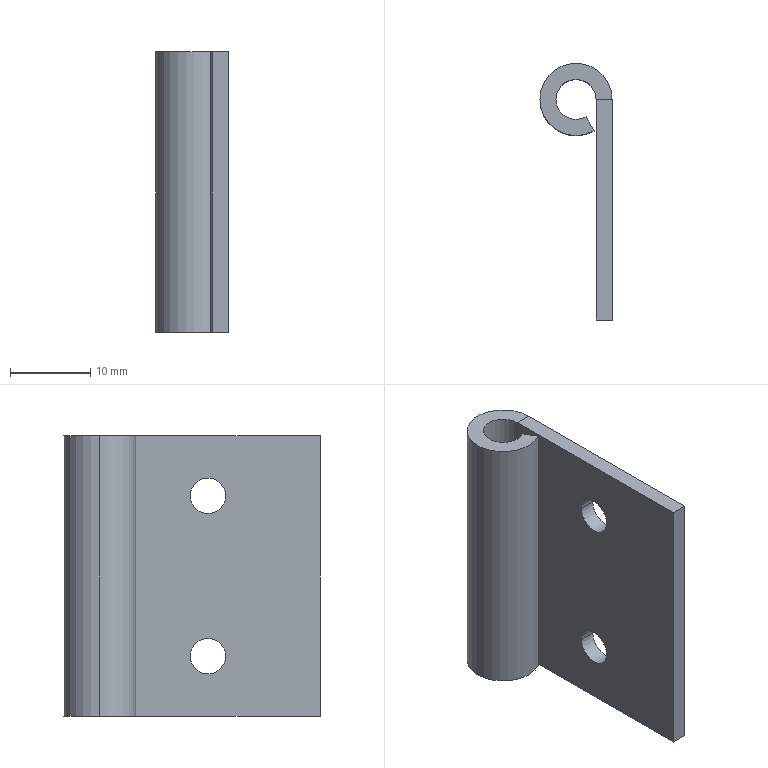Component | SolidWorks | FrontMiddleLowerDoor-1_Hinge(WeldedDoor)-1 | 1 solid | 16 faces | box 9 x 32 x 35 mm | volume 3146 mm3 | cylinder 8 | plane 8 | commonest cylinder face diameters 4.42 x4 9 x2 5 x2
STEP:
#1=CARTESIAN_POINT('',(16.299,14.851,-29.547));
#2=VERTEX_POINT('',#1);
#3=CARTESIAN_POINT('',(16.299,14.677,-29.547));
#4=VERTEX_POINT('',#3);
#5=CARTESIAN_POINT('',(16.299,14.764,-29.547));
#6=DIRECTION('',(1.,0.,-0.));
#7=DIRECTION('',(0.,1.,0.));
#8=AXIS2_PLACEMENT_3D('',#5,#6,#7);
#9=CIRCLE('',#8,0.087);
#10=EDGE_CURVE('',#2,#4,#9,.T.);
#11=ORIENTED_EDGE('',*,*,#10,.F.);
#12=CARTESIAN_POINT('',(16.378,14.851,-29.547));
#13=VERTEX_POINT('',#12);
#14=CARTESIAN_POINT('',(16.299,14.851,-29.547));
#15=DIRECTION('',(1.,0.,-0.));
#16=VECTOR('',#15,39.37);
#17=LINE('',#14,#16);
#18=EDGE_CURVE('',#2,#13,#17,.T.);
#19=ORIENTED_EDGE('',*,*,#18,.T.);
#20=CARTESIAN_POINT('',(16.378,14.677,-29.547));
#21=VERTEX_POINT('',#20);
#22=CARTESIAN_POINT('',(16.378,14.764,-29.547));
#23=DIRECTION('',(1.,0.,-0.));
#24=DIRECTION('',(0.,1.,0.));
#25=AXIS2_PLACEMENT_3D('',#22,#23,#24);
#26=CIRCLE('',#25,0.087);
#27=EDGE_CURVE('',#13,#21,#26,.T.);
#28=ORIENTED_EDGE('',*,*,#27,.T.);
#29=CARTESIAN_POINT('',(16.299,14.677,-29.547));
#30=DIRECTION('',(1.,0.,-0.));
#31=VECTOR('',#30,39.37);
#32=LINE('',#29,#31);
#33=EDGE_CURVE('',#4,#21,#32,.T.);
#34=ORIENTED_EDGE('',*,*,#33,.F.);
#35=EDGE_LOOP('',(#11,#19,#28,#34));
#36=FACE_OUTER_BOUND('',#35,.T.);
#37=CARTESIAN_POINT('',(16.299,14.764,-29.547));
#38=DIRECTION('',(1.,0.,-0.));
#39=DIRECTION('',(0.,-1.,0.));
#40=AXIS2_PLACEMENT_3D('',#37,#38,#39);
#41=CYLINDRICAL_SURFACE('',#40,0.087);
#42=ADVANCED_FACE('',(#36),#41,.F.);
#43=CARTESIAN_POINT('',(16.299,14.851,-30.335));
#44=VERTEX_POINT('',#43);
#45=CARTESIAN_POINT('',(16.299,14.677,-30.335));
#46=VERTEX_POINT('',#45);
#47=CARTESIAN_POINT('',(16.299,14.764,-30.335));
#48=DIRECTION('',(1.,0.,-0.));
#49=DIRECTION('',(0.,-1.,0.));
#50=AXIS2_PLACEMENT_3D('',#47,#48,#49);
#51=CIRCLE('',#50,0.087);
#52=EDGE_CURVE('',#44,#46,#51,.T.);
#53=ORIENTED_EDGE('',*,*,#52,.F.);
#54=CARTESIAN_POINT('',(16.378,14.851,-30.335));
#55=VERTEX_POINT('',#54);
#56=CARTESIAN_POINT('',(16.299,14.851,-30.335));
#57=DIRECTION('',(1.,0.,-0.));
#58=VECTOR('',#57,39.37);
#59=LINE('',#56,#58);
#60=EDGE_CURVE('',#44,#55,#59,.T.);
#61=ORIENTED_EDGE('',*,*,#60,.T.);
#62=CARTESIAN_POINT('',(16.378,14.677,-30.335));
#63=VERTEX_POINT('',#62);
#64=CARTESIAN_POINT('',(16.378,14.764,-30.335));
#65=DIRECTION('',(1.,0.,-0.));
#66=DIRECTION('',(0.,-1.,0.));
#67=AXIS2_PLACEMENT_3D('',#64,#65,#66);
#68=CIRCLE('',#67,0.087);
#69=EDGE_CURVE('',#55,#63,#68,.T.);
#70=ORIENTED_EDGE('',*,*,#69,.T.);
#71=CARTESIAN_POINT('',(16.299,14.677,-30.335));
#72=DIRECTION('',(1.,0.,-0.));
#73=VECTOR('',#72,39.37);
#74=LINE('',#71,#73);
#75=EDGE_CURVE('',#46,#63,#74,.T.);
#76=ORIENTED_EDGE('',*,*,#75,.F.);
#77=EDGE_LOOP('',(#53,#61,#70,#76));
#78=FACE_OUTER_BOUND('',#77,.T.);
#79=CARTESIAN_POINT('',(16.299,14.764,-30.335));
#80=DIRECTION('',(1.,0.,-0.));
#81=DIRECTION('',(0.,-1.,0.));
#82=AXIS2_PLACEMENT_3D('',#79,#80,#81);
#83=CYLINDRICAL_SURFACE('',#82,0.087);
#84=ADVANCED_FACE('',(#78),#83,.F.);
#85=CARTESIAN_POINT('',(16.024,15.295,-30.63));
#86=VERTEX_POINT('',#85);
#87=CARTESIAN_POINT('',(16.378,15.295,-30.63));
#88=VERTEX_POINT('',#87);
#89=CARTESIAN_POINT('',(16.201,15.295,-30.63));
#90=DIRECTION('',(-0.,-0.,-1.));
#91=DIRECTION('',(1.,0.,0.));
#92=AXIS2_PLACEMENT_3D('',#89,#90,#91);
#93=CIRCLE('',#92,0.1772);
#94=EDGE_CURVE('',#86,#88,#93,.T.);
#95=ORIENTED_EDGE('',*,*,#94,.F.);
#96=CARTESIAN_POINT('',(16.024,15.295,-29.252));
#97=VERTEX_POINT('',#96);
#98=CARTESIAN_POINT('',(16.024,15.295,-30.63));
#99=DIRECTION('',(0.,0.,1.));
#100=VECTOR('',#99,39.37);
#101=LINE('',#98,#100);
#102=EDGE_CURVE('',#86,#97,#101,.T.);
#103=ORIENTED_EDGE('',*,*,#102,.T.);
#104=CARTESIAN_POINT('',(16.378,15.295,-29.252));
#105=VERTEX_POINT('',#104);
#106=CARTESIAN_POINT('',(16.201,15.295,-29.252));
#107=DIRECTION('',(-0.,-0.,-1.));
#108=DIRECTION('',(1.,0.,0.));
#109=AXIS2_PLACEMENT_3D('',#106,#107,#108);
#110=CIRCLE('',#109,0.1772);
#111=EDGE_CURVE('',#97,#105,#110,.T.);
#112=ORIENTED_EDGE('',*,*,#111,.T.);
#113=CARTESIAN_POINT('',(16.378,15.295,-30.63));
#114=DIRECTION('',(0.,0.,1.));
#115=VECTOR('',#114,39.37);
#116=LINE('',#113,#115);
#117=EDGE_CURVE('',#88,#105,#116,.T.);
#118=ORIENTED_EDGE('',*,*,#117,.F.);
#119=EDGE_LOOP('',(#95,#103,#112,#118));
#120=FACE_OUTER_BOUND('',#119,.T.);
#121=CARTESIAN_POINT('',(16.201,15.295,-30.63));
#122=DIRECTION('',(0.,0.,1.));
#123=DIRECTION('',(-1.,0.,0.));
#124=AXIS2_PLACEMENT_3D('',#121,#122,#123);
#125=CYLINDRICAL_SURFACE('',#124,0.1772);
#126=ADVANCED_FACE('',(#120),#125,.T.);
#127=CARTESIAN_POINT('',(16.25,15.21,-30.63));
#128=VERTEX_POINT('',#127);
#129=CARTESIAN_POINT('',(16.102,15.295,-30.63));
#130=VERTEX_POINT('',#129);
#131=CARTESIAN_POINT('',(16.201,15.295,-30.63));
#132=DIRECTION('',(-0.,-0.,-1.));
#133=DIRECTION('',(1.,0.,0.));
#134=AXIS2_PLACEMENT_3D('',#131,#132,#133);
#135=CIRCLE('',#134,0.09843);
#136=EDGE_CURVE('',#128,#130,#135,.T.);
#137=ORIENTED_EDGE('',*,*,#136,.T.);
#138=CARTESIAN_POINT('',(16.102,15.295,-29.252));
#139=VERTEX_POINT('',#138);
#140=CARTESIAN_POINT('',(16.102,15.295,-30.63));
#141=DIRECTION('',(0.,0.,1.));
#142=VECTOR('',#141,39.37);
#143=LINE('',#140,#142);
#144=EDGE_CURVE('',#130,#139,#143,.T.);
#145=ORIENTED_EDGE('',*,*,#144,.T.);
#146=CARTESIAN_POINT('',(16.25,15.21,-29.252));
#147=VERTEX_POINT('',#146);
#148=CARTESIAN_POINT('',(16.201,15.295,-29.252));
#149=DIRECTION('',(-0.,-0.,-1.));
#150=DIRECTION('',(1.,0.,0.));
#151=AXIS2_PLACEMENT_3D('',#148,#149,#150);
#152=CIRCLE('',#151,0.09843);
#153=EDGE_CURVE('',#147,#139,#152,.T.);
#154=ORIENTED_EDGE('',*,*,#153,.F.);
#155=CARTESIAN_POINT('',(16.25,15.21,-30.63));
#156=DIRECTION('',(0.,0.,1.));
#157=VECTOR('',#156,39.37);
#158=LINE('',#155,#157);
#159=EDGE_CURVE('',#128,#147,#158,.T.);
#160=ORIENTED_EDGE('',*,*,#159,.F.);
#161=EDGE_LOOP('',(#137,#145,#154,#160));
#162=FACE_OUTER_BOUND('',#161,.T.);
#163=CARTESIAN_POINT('',(16.201,15.295,-30.63));
#164=DIRECTION('',(0.,0.,1.));
#165=DIRECTION('',(-1.,0.,0.));
#166=AXIS2_PLACEMENT_3D('',#163,#164,#165);
#167=CYLINDRICAL_SURFACE('',#166,0.09843);
#168=ADVANCED_FACE('',(#162),#167,.F.);
#169=CARTESIAN_POINT('',(16.299,15.295,-30.63));
#170=VERTEX_POINT('',#169);
#171=CARTESIAN_POINT('',(16.299,15.295,-30.63));
#172=DIRECTION('',(1.,0.,-0.));
#173=VECTOR('',#172,39.37);
#174=LINE('',#171,#173);
#175=EDGE_CURVE('',#170,#88,#174,.T.);
#176=ORIENTED_EDGE('',*,*,#175,.F.);
#177=CARTESIAN_POINT('',(16.201,15.295,-30.63));
#178=DIRECTION('',(-0.,-0.,-1.));
#179=DIRECTION('',(1.,0.,0.));
#180=AXIS2_PLACEMENT_3D('',#177,#178,#179);
#181=CIRCLE('',#180,0.09843);
#182=EDGE_CURVE('',#130,#170,#181,.T.);
#183=ORIENTED_EDGE('',*,*,#182,.F.);
#184=ORIENTED_EDGE('',*,*,#136,.F.);
#185=CARTESIAN_POINT('',(16.289,15.142,-30.63));
#186=VERTEX_POINT('',#185);
#187=CARTESIAN_POINT('',(16.289,15.142,-30.63));
#188=DIRECTION('',(-0.5,0.866,0.));
#189=VECTOR('',#188,39.37);
#190=LINE('',#187,#189);
#191=EDGE_CURVE('',#186,#128,#190,.T.);
#192=ORIENTED_EDGE('',*,*,#191,.F.);
#193=CARTESIAN_POINT('',(16.201,15.295,-30.63));
#194=DIRECTION('',(-0.,-0.,-1.));
#195=DIRECTION('',(1.,0.,0.));
#196=AXIS2_PLACEMENT_3D('',#193,#194,#195);
#197=CIRCLE('',#196,0.1772);
#198=EDGE_CURVE('',#186,#86,#197,.T.);
#199=ORIENTED_EDGE('',*,*,#198,.T.);
#200=ORIENTED_EDGE('',*,*,#94,.T.);
#201=EDGE_LOOP('',(#176,#183,#184,#192,#199,#200));
#202=FACE_OUTER_BOUND('',#201,.T.);
#203=CARTESIAN_POINT('',(16.299,15.295,-30.63));
#204=DIRECTION('',(-0.,-0.,-1.));
#205=DIRECTION('',(1.,0.,-0.));
#206=AXIS2_PLACEMENT_3D('',#203,#204,#205);
#207=PLANE('',#206);
#208=ADVANCED_FACE('',(#202),#207,.T.);
#209=CARTESIAN_POINT('',(16.299,15.295,-29.252));
#210=VERTEX_POINT('',#209);
#211=CARTESIAN_POINT('',(16.378,15.295,-29.252));
#212=DIRECTION('',(-1.,-0.,0.));
#213=VECTOR('',#212,39.37);
#214=LINE('',#211,#213);
#215=EDGE_CURVE('',#105,#210,#214,.T.);
#216=ORIENTED_EDGE('',*,*,#215,.F.);
#217=ORIENTED_EDGE('',*,*,#111,.F.);
#218=CARTESIAN_POINT('',(16.289,15.142,-29.252));
#219=VERTEX_POINT('',#218);
#220=CARTESIAN_POINT('',(16.201,15.295,-29.252));
#221=DIRECTION('',(-0.,-0.,-1.));
#222=DIRECTION('',(1.,0.,0.));
#223=AXIS2_PLACEMENT_3D('',#220,#221,#222);
#224=CIRCLE('',#223,0.1772);
#225=EDGE_CURVE('',#219,#97,#224,.T.);
#226=ORIENTED_EDGE('',*,*,#225,.F.);
#227=CARTESIAN_POINT('',(16.289,15.142,-29.252));
#228=DIRECTION('',(-0.5,0.866,0.));
#229=VECTOR('',#228,39.37);
#230=LINE('',#227,#229);
#231=EDGE_CURVE('',#219,#147,#230,.T.);
#232=ORIENTED_EDGE('',*,*,#231,.T.);
#233=ORIENTED_EDGE('',*,*,#153,.T.);
#234=CARTESIAN_POINT('',(16.201,15.295,-29.252));
#235=DIRECTION('',(-0.,-0.,-1.));
#236=DIRECTION('',(1.,0.,0.));
#237=AXIS2_PLACEMENT_3D('',#234,#235,#236);
#238=CIRCLE('',#237,0.09843);
#239=EDGE_CURVE('',#139,#210,#238,.T.);
#240=ORIENTED_EDGE('',*,*,#239,.T.);
#241=EDGE_LOOP('',(#216,#217,#226,#232,#233,#240));
#242=FACE_OUTER_BOUND('',#241,.T.);
#243=CARTESIAN_POINT('',(16.378,15.295,-29.252));
#244=DIRECTION('',(0.,0.,1.));
#245=DIRECTION('',(-1.,-0.,0.));
#246=AXIS2_PLACEMENT_3D('',#243,#244,#245);
#247=PLANE('',#246);
#248=ADVANCED_FACE('',(#242),#247,.T.);
#249=CARTESIAN_POINT('',(16.378,14.764,-29.547));
#250=DIRECTION('',(1.,0.,-0.));
#251=DIRECTION('',(0.,1.,0.));
#252=AXIS2_PLACEMENT_3D('',#249,#250,#251);
#253=CIRCLE('',#252,0.087);
#254=EDGE_CURVE('',#21,#13,#253,.T.);
#255=ORIENTED_EDGE('',*,*,#254,.F.);
#256=ORIENTED_EDGE('',*,*,#27,.F.);
#257=EDGE_LOOP('',(#255,#256));
#258=FACE_BOUND('',#257,.T.);
#259=CARTESIAN_POINT('',(16.378,14.764,-30.335));
#260=DIRECTION('',(1.,0.,-0.));
#261=DIRECTION('',(0.,-1.,0.));
#262=AXIS2_PLACEMENT_3D('',#259,#260,#261);
#263=CIRCLE('',#262,0.087);
#264=EDGE_CURVE('',#63,#55,#263,.T.);
#265=ORIENTED_EDGE('',*,*,#264,.F.);
#266=ORIENTED_EDGE('',*,*,#69,.F.);
#267=EDGE_LOOP('',(#265,#266));
#268=FACE_BOUND('',#267,.T.);
#269=CARTESIAN_POINT('',(16.378,14.213,-29.252));
#270=VERTEX_POINT('',#269);
#271=CARTESIAN_POINT('',(16.378,15.295,-29.252));
#272=DIRECTION('',(0.,-1.,0.));
#273=VECTOR('',#272,39.37);
#274=LINE('',#271,#273);
#275=EDGE_CURVE('',#105,#270,#274,.T.);
#276=ORIENTED_EDGE('',*,*,#275,.T.);
#277=CARTESIAN_POINT('',(16.378,14.213,-30.63));
#278=VERTEX_POINT('',#277);
#279=CARTESIAN_POINT('',(16.378,14.213,-30.63));
#280=DIRECTION('',(0.,0.,1.));
#281=VECTOR('',#280,39.37);
#282=LINE('',#279,#281);
#283=EDGE_CURVE('',#278,#270,#282,.T.);
#284=ORIENTED_EDGE('',*,*,#283,.F.);
#285=CARTESIAN_POINT('',(16.378,15.295,-30.63));
#286=DIRECTION('',(0.,-1.,0.));
#287=VECTOR('',#286,39.37);
#288=LINE('',#285,#287);
#289=EDGE_CURVE('',#88,#278,#288,.T.);
#290=ORIENTED_EDGE('',*,*,#289,.F.);
#291=ORIENTED_EDGE('',*,*,#117,.T.);
#292=EDGE_LOOP('',(#276,#284,#290,#291));
#293=FACE_OUTER_BOUND('',#292,.T.);
#294=CARTESIAN_POINT('',(16.378,15.295,-30.63));
#295=DIRECTION('',(-1.,-0.,0.));
#296=DIRECTION('',(-0.,1.,-0.));
#297=AXIS2_PLACEMENT_3D('',#294,#295,#296);
#298=PLANE('',#297);
#299=ADVANCED_FACE('',(#258,#268,#293),#298,.F.);
#300=CARTESIAN_POINT('',(16.299,14.213,-29.252));
#301=VERTEX_POINT('',#300);
#302=CARTESIAN_POINT('',(16.299,14.213,-29.252));
#303=DIRECTION('',(1.,0.,-0.));
#304=VECTOR('',#303,39.37);
#305=LINE('',#302,#304);
#306=EDGE_CURVE('',#301,#270,#305,.T.);
#307=ORIENTED_EDGE('',*,*,#306,.F.);
#308=CARTESIAN_POINT('',(16.299,14.213,-30.63));
#309=VERTEX_POINT('',#308);
#310=CARTESIAN_POINT('',(16.299,14.213,-30.63));
#311=DIRECTION('',(0.,0.,1.));
#312=VECTOR('',#311,39.37);
#313=LINE('',#310,#312);
#314=EDGE_CURVE('',#309,#301,#313,.T.);
#315=ORIENTED_EDGE('',*,*,#314,.F.);
#316=CARTESIAN_POINT('',(16.299,14.213,-30.63));
#317=DIRECTION('',(1.,0.,-0.));
#318=VECTOR('',#317,39.37);
#319=LINE('',#316,#318);
#320=EDGE_CURVE('',#309,#278,#319,.T.);
#321=ORIENTED_EDGE('',*,*,#320,.T.);
#322=ORIENTED_EDGE('',*,*,#283,.T.);
#323=EDGE_LOOP('',(#307,#315,#321,#322));
#324=FACE_OUTER_BOUND('',#323,.T.);
#325=CARTESIAN_POINT('',(16.299,14.213,-30.63));
#326=DIRECTION('',(0.,-1.,0.));
#327=DIRECTION('',(-0.,-0.,-1.));
#328=AXIS2_PLACEMENT_3D('',#325,#326,#327);
#329=PLANE('',#328);
#330=ADVANCED_FACE('',(#324),#329,.T.);
#331=CARTESIAN_POINT('',(16.299,14.764,-29.547));
#332=DIRECTION('',(1.,0.,-0.));
#333=DIRECTION('',(0.,1.,0.));
#334=AXIS2_PLACEMENT_3D('',#331,#332,#333);
#335=CIRCLE('',#334,0.087);
#336=EDGE_CURVE('',#4,#2,#335,.T.);
#337=ORIENTED_EDGE('',*,*,#336,.T.);
#338=ORIENTED_EDGE('',*,*,#10,.T.);
#339=EDGE_LOOP('',(#337,#338));
#340=FACE_BOUND('',#339,.T.);
#341=CARTESIAN_POINT('',(16.299,14.764,-30.335));
#342=DIRECTION('',(1.,0.,-0.));
#343=DIRECTION('',(0.,-1.,0.));
#344=AXIS2_PLACEMENT_3D('',#341,#342,#343);
#345=CIRCLE('',#344,0.087);
#346=EDGE_CURVE('',#46,#44,#345,.T.);
#347=ORIENTED_EDGE('',*,*,#346,.T.);
#348=ORIENTED_EDGE('',*,*,#52,.T.);
#349=EDGE_LOOP('',(#347,#348));
#350=FACE_BOUND('',#349,.T.);
#351=CARTESIAN_POINT('',(16.299,15.295,-29.252));
#352=DIRECTION('',(0.,-1.,0.));
#353=VECTOR('',#352,39.37);
#354=LINE('',#351,#353);
#355=EDGE_CURVE('',#210,#301,#354,.T.);
#356=ORIENTED_EDGE('',*,*,#355,.F.);
#357=CARTESIAN_POINT('',(16.299,15.295,-30.63));
#358=DIRECTION('',(0.,0.,1.));
#359=VECTOR('',#358,39.37);
#360=LINE('',#357,#359);
#361=EDGE_CURVE('',#170,#210,#360,.T.);
#362=ORIENTED_EDGE('',*,*,#361,.F.);
#363=CARTESIAN_POINT('',(16.299,15.295,-30.63));
#364=DIRECTION('',(0.,-1.,0.));
#365=VECTOR('',#364,39.37);
#366=LINE('',#363,#365);
#367=EDGE_CURVE('',#170,#309,#366,.T.);
#368=ORIENTED_EDGE('',*,*,#367,.T.);
#369=ORIENTED_EDGE('',*,*,#314,.T.);
#370=EDGE_LOOP('',(#356,#362,#368,#369));
#371=FACE_OUTER_BOUND('',#370,.T.);
#372=CARTESIAN_POINT('',(16.299,15.295,-30.63));
#373=DIRECTION('',(-1.,-0.,0.));
#374=DIRECTION('',(-0.,1.,-0.));
#375=AXIS2_PLACEMENT_3D('',#372,#373,#374);
#376=PLANE('',#375);
#377=ADVANCED_FACE('',(#340,#350,#371),#376,.T.);
#378=ORIENTED_EDGE('',*,*,#144,.F.);
#379=ORIENTED_EDGE('',*,*,#182,.T.);
#380=ORIENTED_EDGE('',*,*,#361,.T.);
#381=ORIENTED_EDGE('',*,*,#239,.F.);
#382=EDGE_LOOP('',(#378,#379,#380,#381));
#383=FACE_OUTER_BOUND('',#382,.T.);
#384=CARTESIAN_POINT('',(16.201,15.295,-30.63));
#385=DIRECTION('',(0.,0.,1.));
#386=DIRECTION('',(-1.,0.,0.));
#387=AXIS2_PLACEMENT_3D('',#384,#385,#386);
#388=CYLINDRICAL_SURFACE('',#387,0.09843);
#389=ADVANCED_FACE('',(#383),#388,.F.);
#390=ORIENTED_EDGE('',*,*,#231,.F.);
#391=CARTESIAN_POINT('',(16.289,15.142,-30.63));
#392=DIRECTION('',(0.,0.,1.));
#393=VECTOR('',#392,39.37);
#394=LINE('',#391,#393);
#395=EDGE_CURVE('',#186,#219,#394,.T.);
#396=ORIENTED_EDGE('',*,*,#395,.F.);
#397=ORIENTED_EDGE('',*,*,#191,.T.);
#398=ORIENTED_EDGE('',*,*,#159,.T.);
#399=EDGE_LOOP('',(#390,#396,#397,#398));
#400=FACE_OUTER_BOUND('',#399,.T.);
#401=CARTESIAN_POINT('',(16.289,15.142,-30.63));
#402=DIRECTION('',(0.866,0.5,-0.));
#403=DIRECTION('',(0.5,-0.866,-0.));
#404=AXIS2_PLACEMENT_3D('',#401,#402,#403);
#405=PLANE('',#404);
#406=ADVANCED_FACE('',(#400),#405,.T.);
#407=ORIENTED_EDGE('',*,*,#102,.F.);
#408=ORIENTED_EDGE('',*,*,#198,.F.);
#409=ORIENTED_EDGE('',*,*,#395,.T.);
#410=ORIENTED_EDGE('',*,*,#225,.T.);
#411=EDGE_LOOP('',(#407,#408,#409,#410));
#412=FACE_OUTER_BOUND('',#411,.T.);
#413=CARTESIAN_POINT('',(16.201,15.295,-30.63));
#414=DIRECTION('',(0.,0.,1.));
#415=DIRECTION('',(-1.,0.,0.));
#416=AXIS2_PLACEMENT_3D('',#413,#414,#415);
#417=CYLINDRICAL_SURFACE('',#416,0.1772);
#418=ADVANCED_FACE('',(#412),#417,.T.);
#419=ORIENTED_EDGE('',*,*,#289,.T.);
#420=ORIENTED_EDGE('',*,*,#320,.F.);
#421=ORIENTED_EDGE('',*,*,#367,.F.);
#422=ORIENTED_EDGE('',*,*,#175,.T.);
#423=EDGE_LOOP('',(#419,#420,#421,#422));
#424=FACE_OUTER_BOUND('',#423,.T.);
#425=CARTESIAN_POINT('',(16.201,15.295,-30.63));
#426=DIRECTION('',(-0.,-0.,-1.));
#427=DIRECTION('',(1.,0.,-0.));
#428=AXIS2_PLACEMENT_3D('',#425,#426,#427);
#429=PLANE('',#428);
#430=ADVANCED_FACE('',(#424),#429,.T.);
#431=ORIENTED_EDGE('',*,*,#275,.F.);
#432=ORIENTED_EDGE('',*,*,#215,.T.);
#433=ORIENTED_EDGE('',*,*,#355,.T.);
#434=ORIENTED_EDGE('',*,*,#306,.T.);
#435=EDGE_LOOP('',(#431,#432,#433,#434));
#436=FACE_OUTER_BOUND('',#435,.T.);
#437=CARTESIAN_POINT('',(16.201,15.295,-29.252));
#438=DIRECTION('',(-0.,-0.,-1.));
#439=DIRECTION('',(1.,0.,-0.));
#440=AXIS2_PLACEMENT_3D('',#437,#438,#439);
#441=PLANE('',#440);
#442=ADVANCED_FACE('',(#436),#441,.F.);
#443=ORIENTED_EDGE('',*,*,#60,.F.);
#444=ORIENTED_EDGE('',*,*,#346,.F.);
#445=ORIENTED_EDGE('',*,*,#75,.T.);
#446=ORIENTED_EDGE('',*,*,#264,.T.);
#447=EDGE_LOOP('',(#443,#444,#445,#446));
#448=FACE_OUTER_BOUND('',#447,.T.);
#449=CARTESIAN_POINT('',(16.299,14.764,-30.335));
#450=DIRECTION('',(1.,0.,-0.));
#451=DIRECTION('',(0.,-1.,0.));
#452=AXIS2_PLACEMENT_3D('',#449,#450,#451);
#453=CYLINDRICAL_SURFACE('',#452,0.087);
#454=ADVANCED_FACE('',(#448),#453,.F.);
#455=ORIENTED_EDGE('',*,*,#18,.F.);
#456=ORIENTED_EDGE('',*,*,#336,.F.);
#457=ORIENTED_EDGE('',*,*,#33,.T.);
#458=ORIENTED_EDGE('',*,*,#254,.T.);
#459=EDGE_LOOP('',(#455,#456,#457,#458));
#460=FACE_OUTER_BOUND('',#459,.T.);
#461=CARTESIAN_POINT('',(16.299,14.764,-29.547));
#462=DIRECTION('',(1.,0.,-0.));
#463=DIRECTION('',(0.,-1.,0.));
#464=AXIS2_PLACEMENT_3D('',#461,#462,#463);
#465=CYLINDRICAL_SURFACE('',#464,0.087);
#466=ADVANCED_FACE('',(#460),#465,.F.);
#467=CLOSED_SHELL('',(#42,#84,#126,#168,#208,#248,#299,#330,#377,#389,#406,#418,#430,#442,#454,#466));
#468=MANIFOLD_SOLID_BREP('',#467);
#469=CARTESIAN_POINT('',(0.,0.,0.));
#470=DIRECTION('',(0.,0.,1.));
#471=DIRECTION('',(1.,0.,0.));
#472=AXIS2_PLACEMENT_3D('',#469,#470,#471);
#473=(LENGTH_UNIT()NAMED_UNIT(*)SI_UNIT($,.METRE.));
#474=LENGTH_MEASURE_WITH_UNIT(LENGTH_MEASURE(0.0254),#473);
#475=DIMENSIONAL_EXPONENTS(1.,0.,0.,0.,0.,0.,0.);
#476=(CONVERSION_BASED_UNIT('',#474)LENGTH_UNIT()NAMED_UNIT(#475));
#477=UNCERTAINTY_MEASURE_WITH_UNIT(LENGTH_MEASURE(0.00001),#476,'','');
#478=(NAMED_UNIT(*)PLANE_ANGLE_UNIT()SI_UNIT($,.RADIAN.));
#479=(NAMED_UNIT(*)SI_UNIT($,.STERADIAN.)SOLID_ANGLE_UNIT());
#480=(GEOMETRIC_REPRESENTATION_CONTEXT(3)GLOBAL_UNCERTAINTY_ASSIGNED_CONTEXT((#477))GLOBAL_UNIT_ASSIGNED_CONTEXT((#476,#478,#479))REPRESENTATION_CONTEXT('',''));
#481=ADVANCED_BREP_SHAPE_REPRESENTATION('',(#468,#472),#480);
#482=COLOUR_RGB('',0.7922,0.8196,0.9333);
#483=FILL_AREA_STYLE_COLOUR('',#482);
#484=FILL_AREA_STYLE('',(#483));
#485=SURFACE_STYLE_FILL_AREA(#484);
#486=SURFACE_SIDE_STYLE('',(#485));
#487=SURFACE_STYLE_USAGE(.BOTH.,#486);
#488=PRESENTATION_STYLE_ASSIGNMENT((#487));
#489=STYLED_ITEM('',(#488),#468);
#490=(LENGTH_UNIT()NAMED_UNIT(*)SI_UNIT($,.METRE.));
#491=LENGTH_MEASURE_WITH_UNIT(LENGTH_MEASURE(0.0254),#490);
#492=DIMENSIONAL_EXPONENTS(1.,0.,0.,0.,0.,0.,0.);
#493=(CONVERSION_BASED_UNIT('',#491)LENGTH_UNIT()NAMED_UNIT(#492));
#494=UNCERTAINTY_MEASURE_WITH_UNIT(LENGTH_MEASURE(0.00001),#493,'','');
#495=(NAMED_UNIT(*)PLANE_ANGLE_UNIT()SI_UNIT($,.RADIAN.));
#496=(NAMED_UNIT(*)SI_UNIT($,.STERADIAN.)SOLID_ANGLE_UNIT());
#497=(GEOMETRIC_REPRESENTATION_CONTEXT(3)GLOBAL_UNCERTAINTY_ASSIGNED_CONTEXT((#494))GLOBAL_UNIT_ASSIGNED_CONTEXT((#493,#495,#496))REPRESENTATION_CONTEXT('',''));
#498=MECHANICAL_DESIGN_GEOMETRIC_PRESENTATION_REPRESENTATION('',(#489),#497);
#499=PRESENTATION_LAYER_ASSIGNMENT('','',(#489));